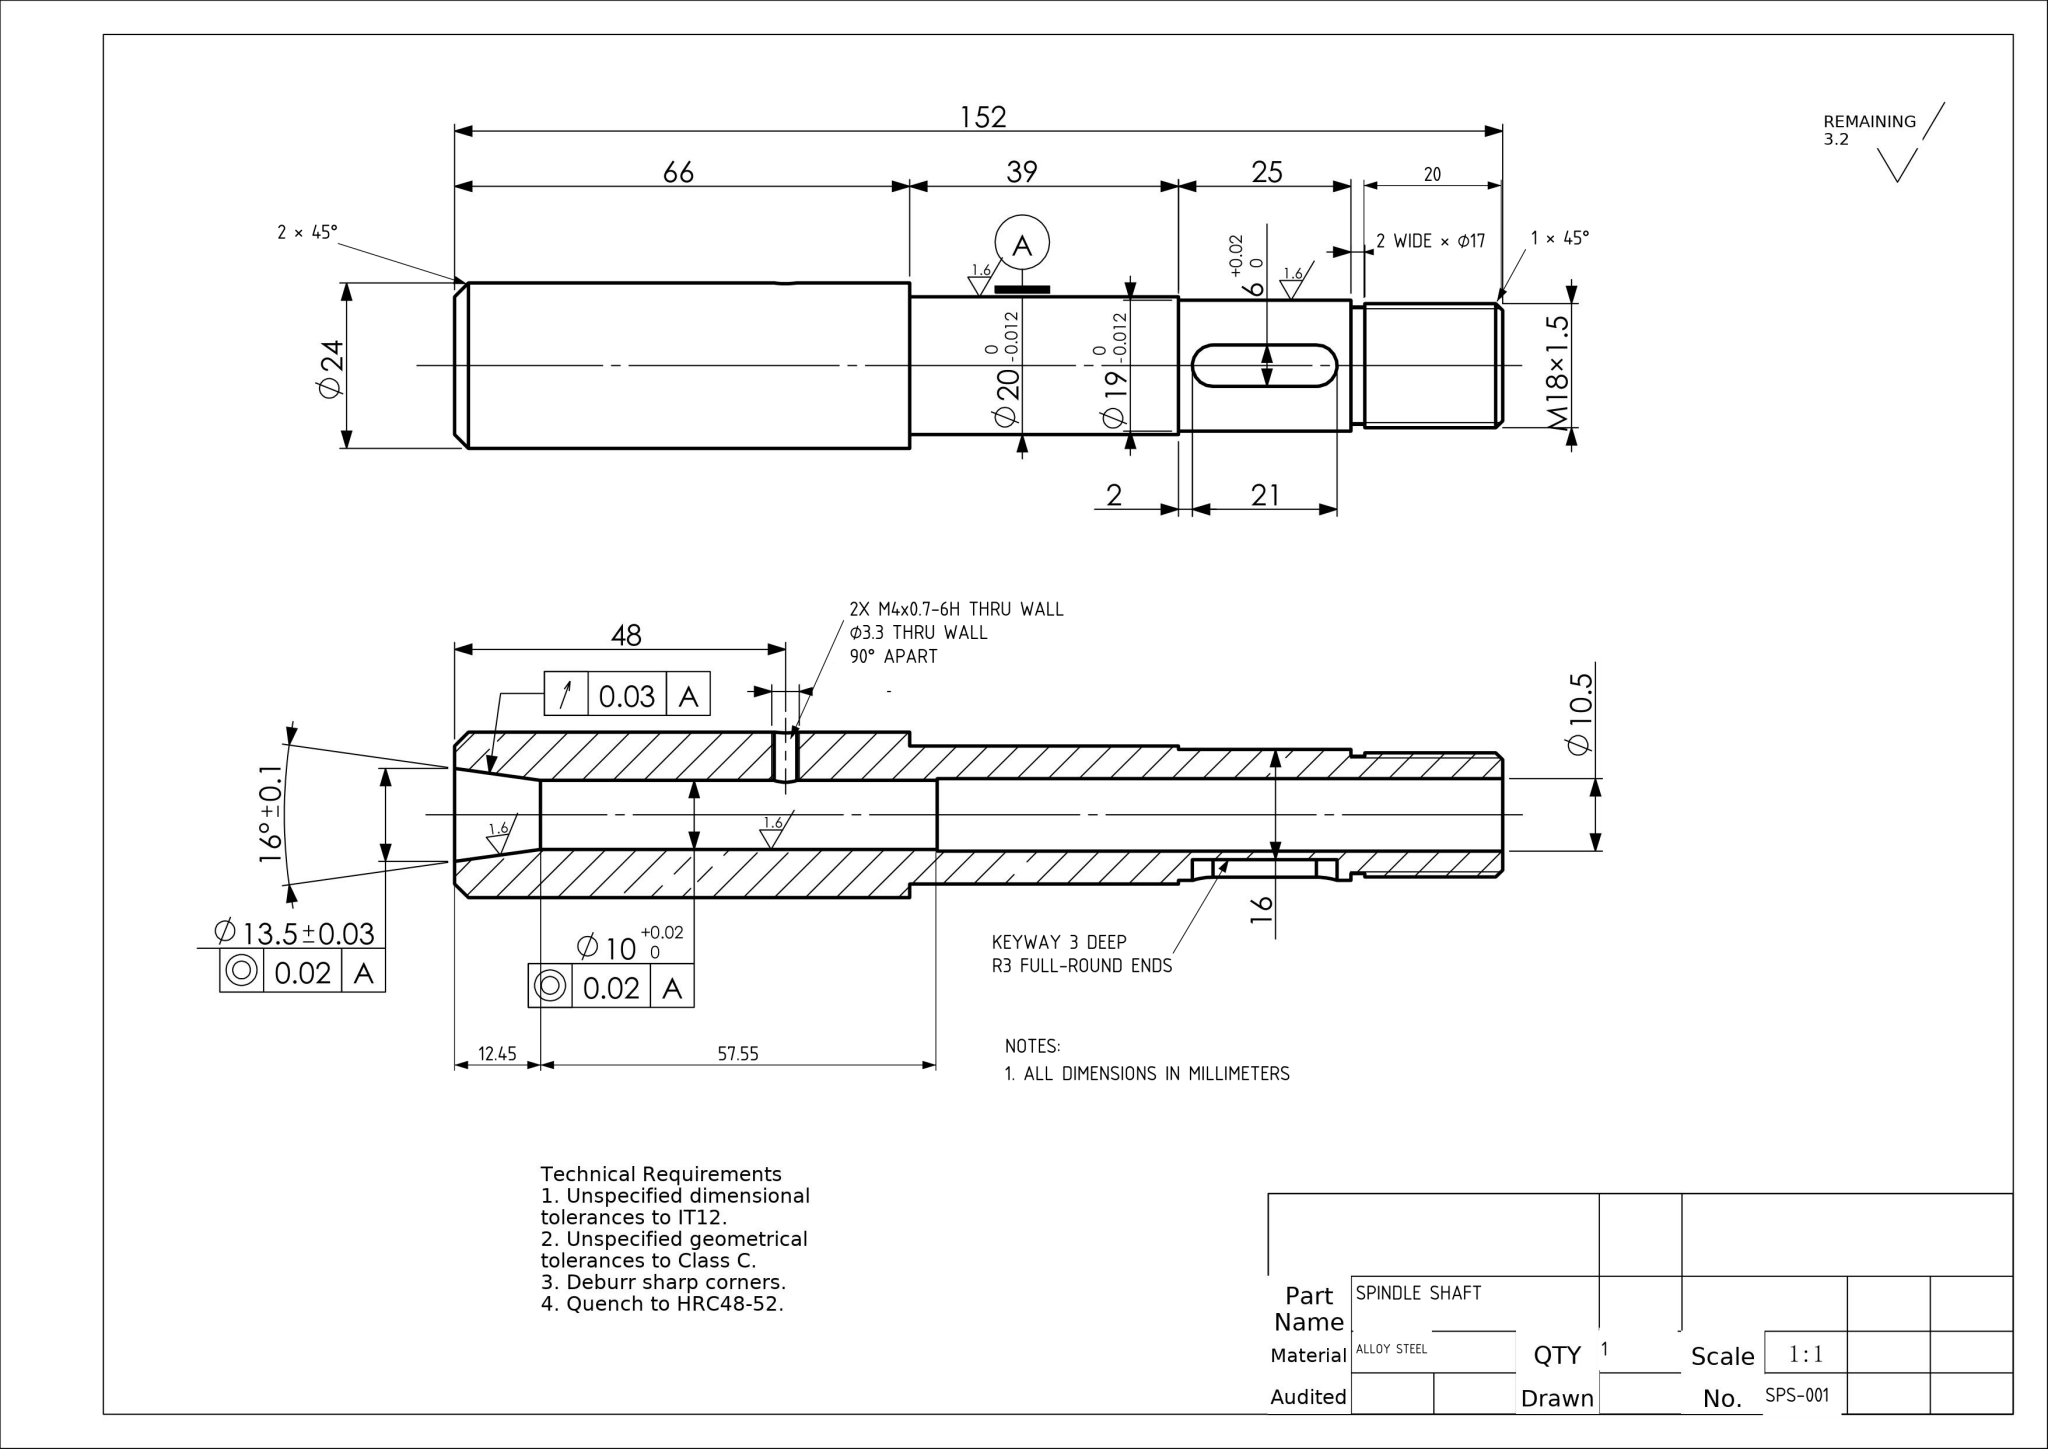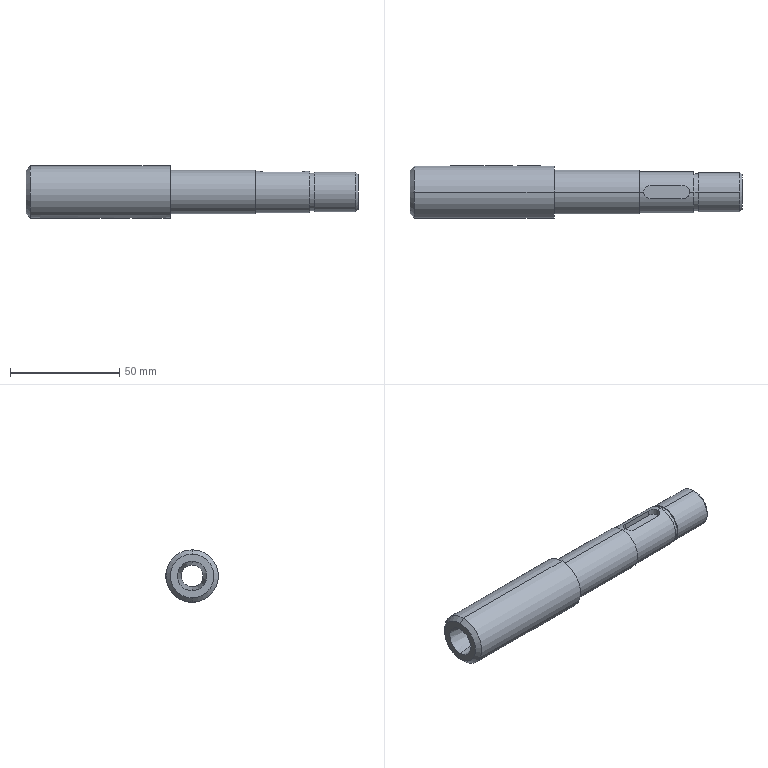Part | NX | mm | 1 solid | 37 faces | box 152 x 24 x 24 mm | volume 41134 mm3 | cylinder 21 | plane 10 | cone 6 | commonest cylinder face diameters 3.3 x4 6 x3 10.5 x2 10 x2 18 x2 17 x2 20 x2 24 x2